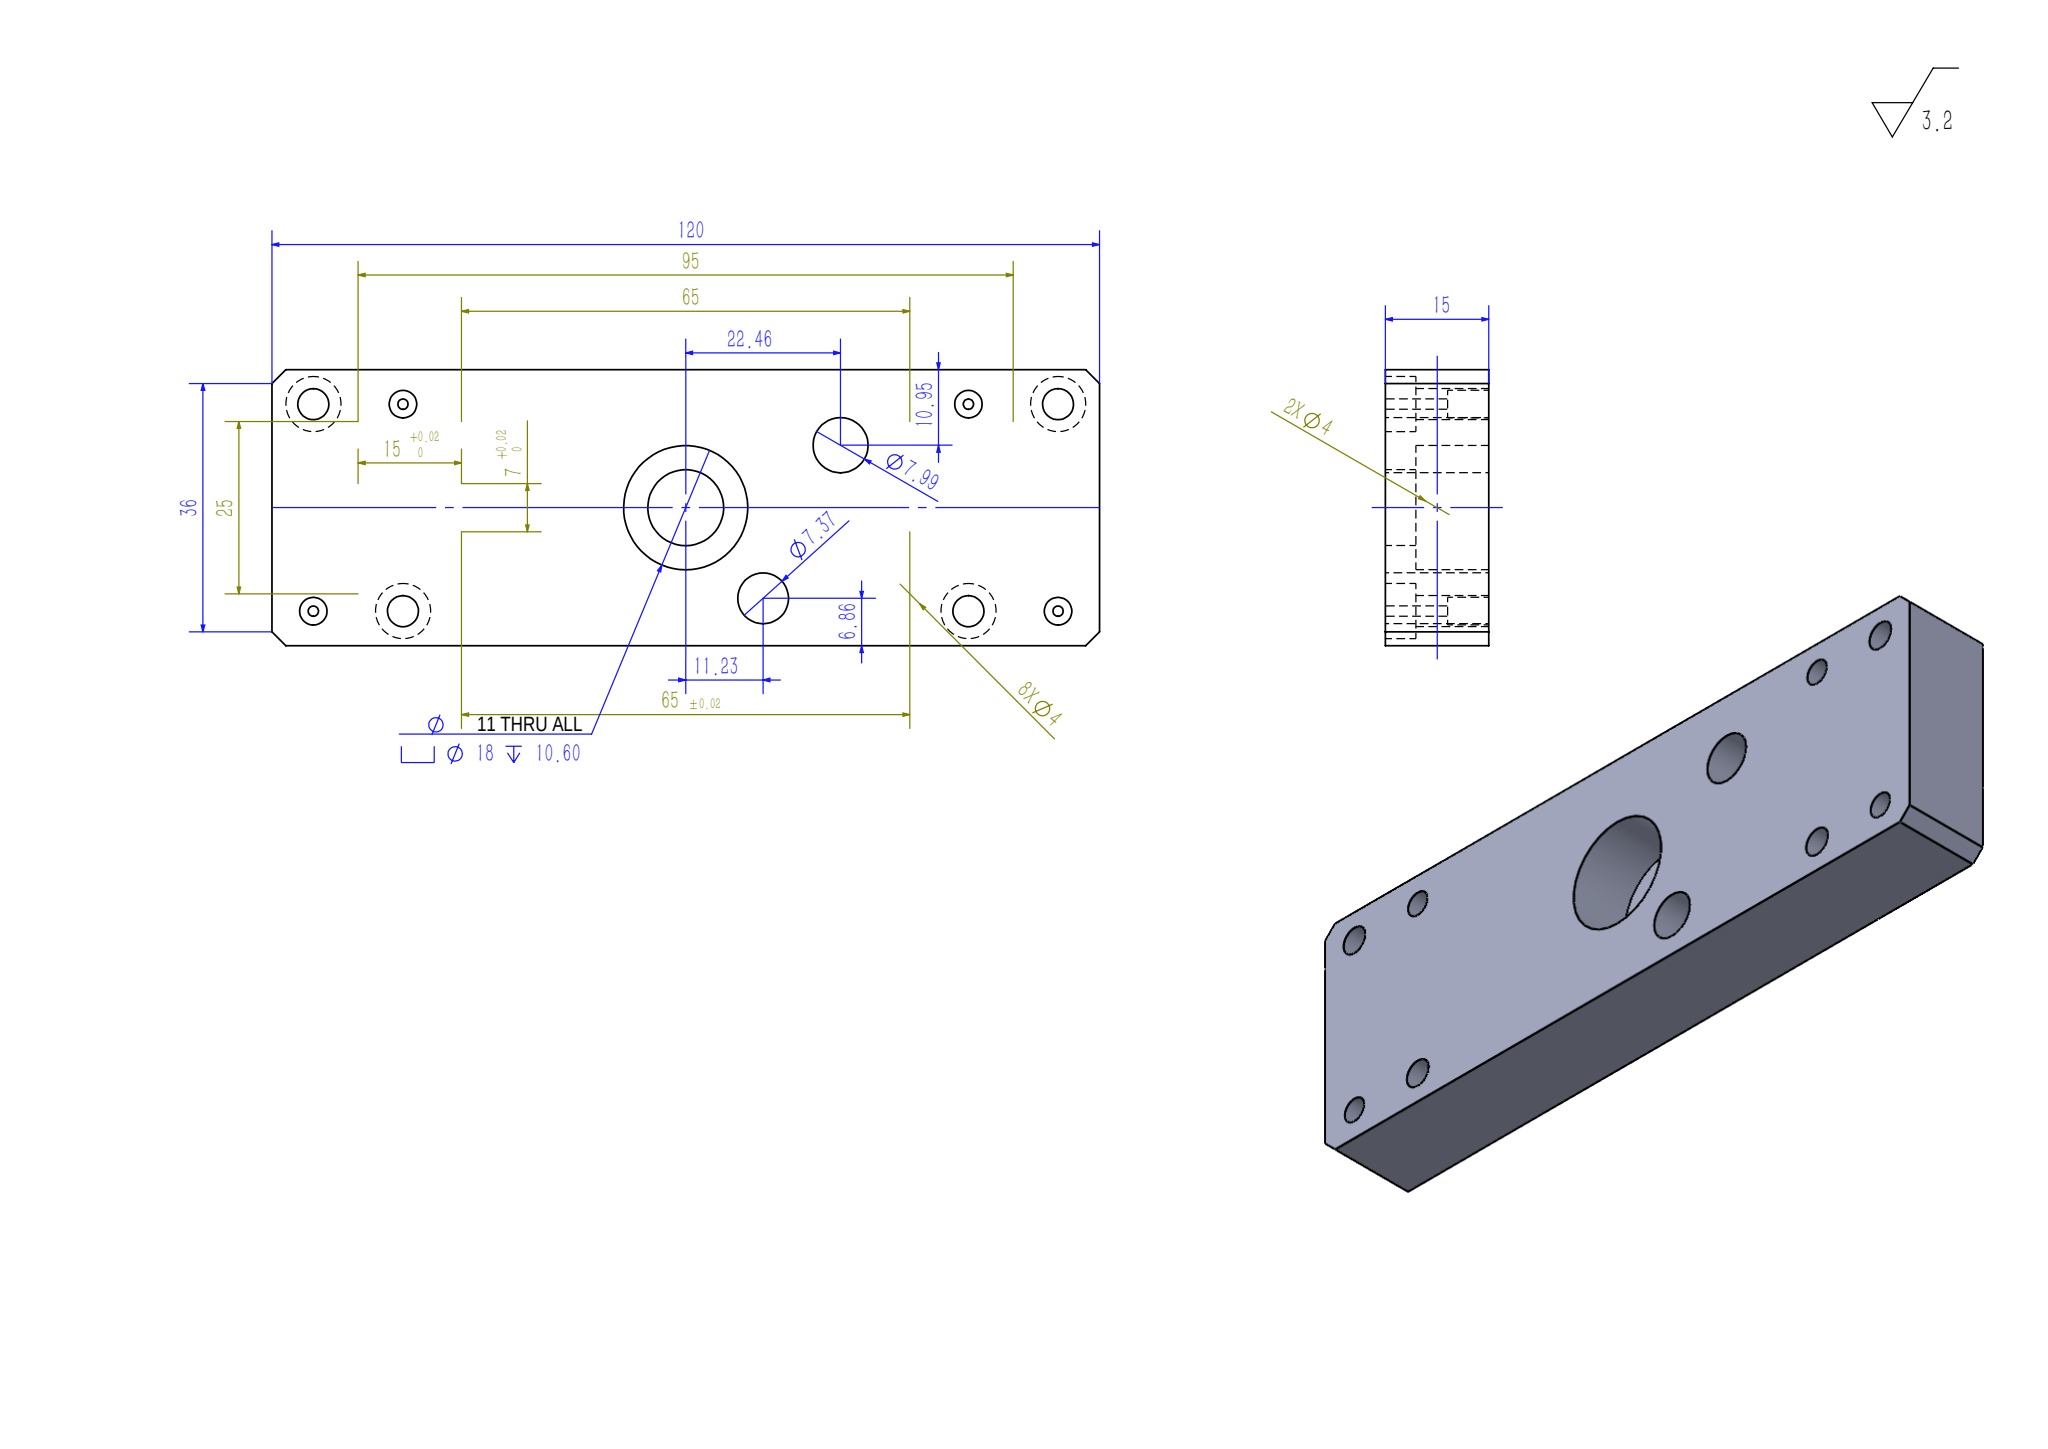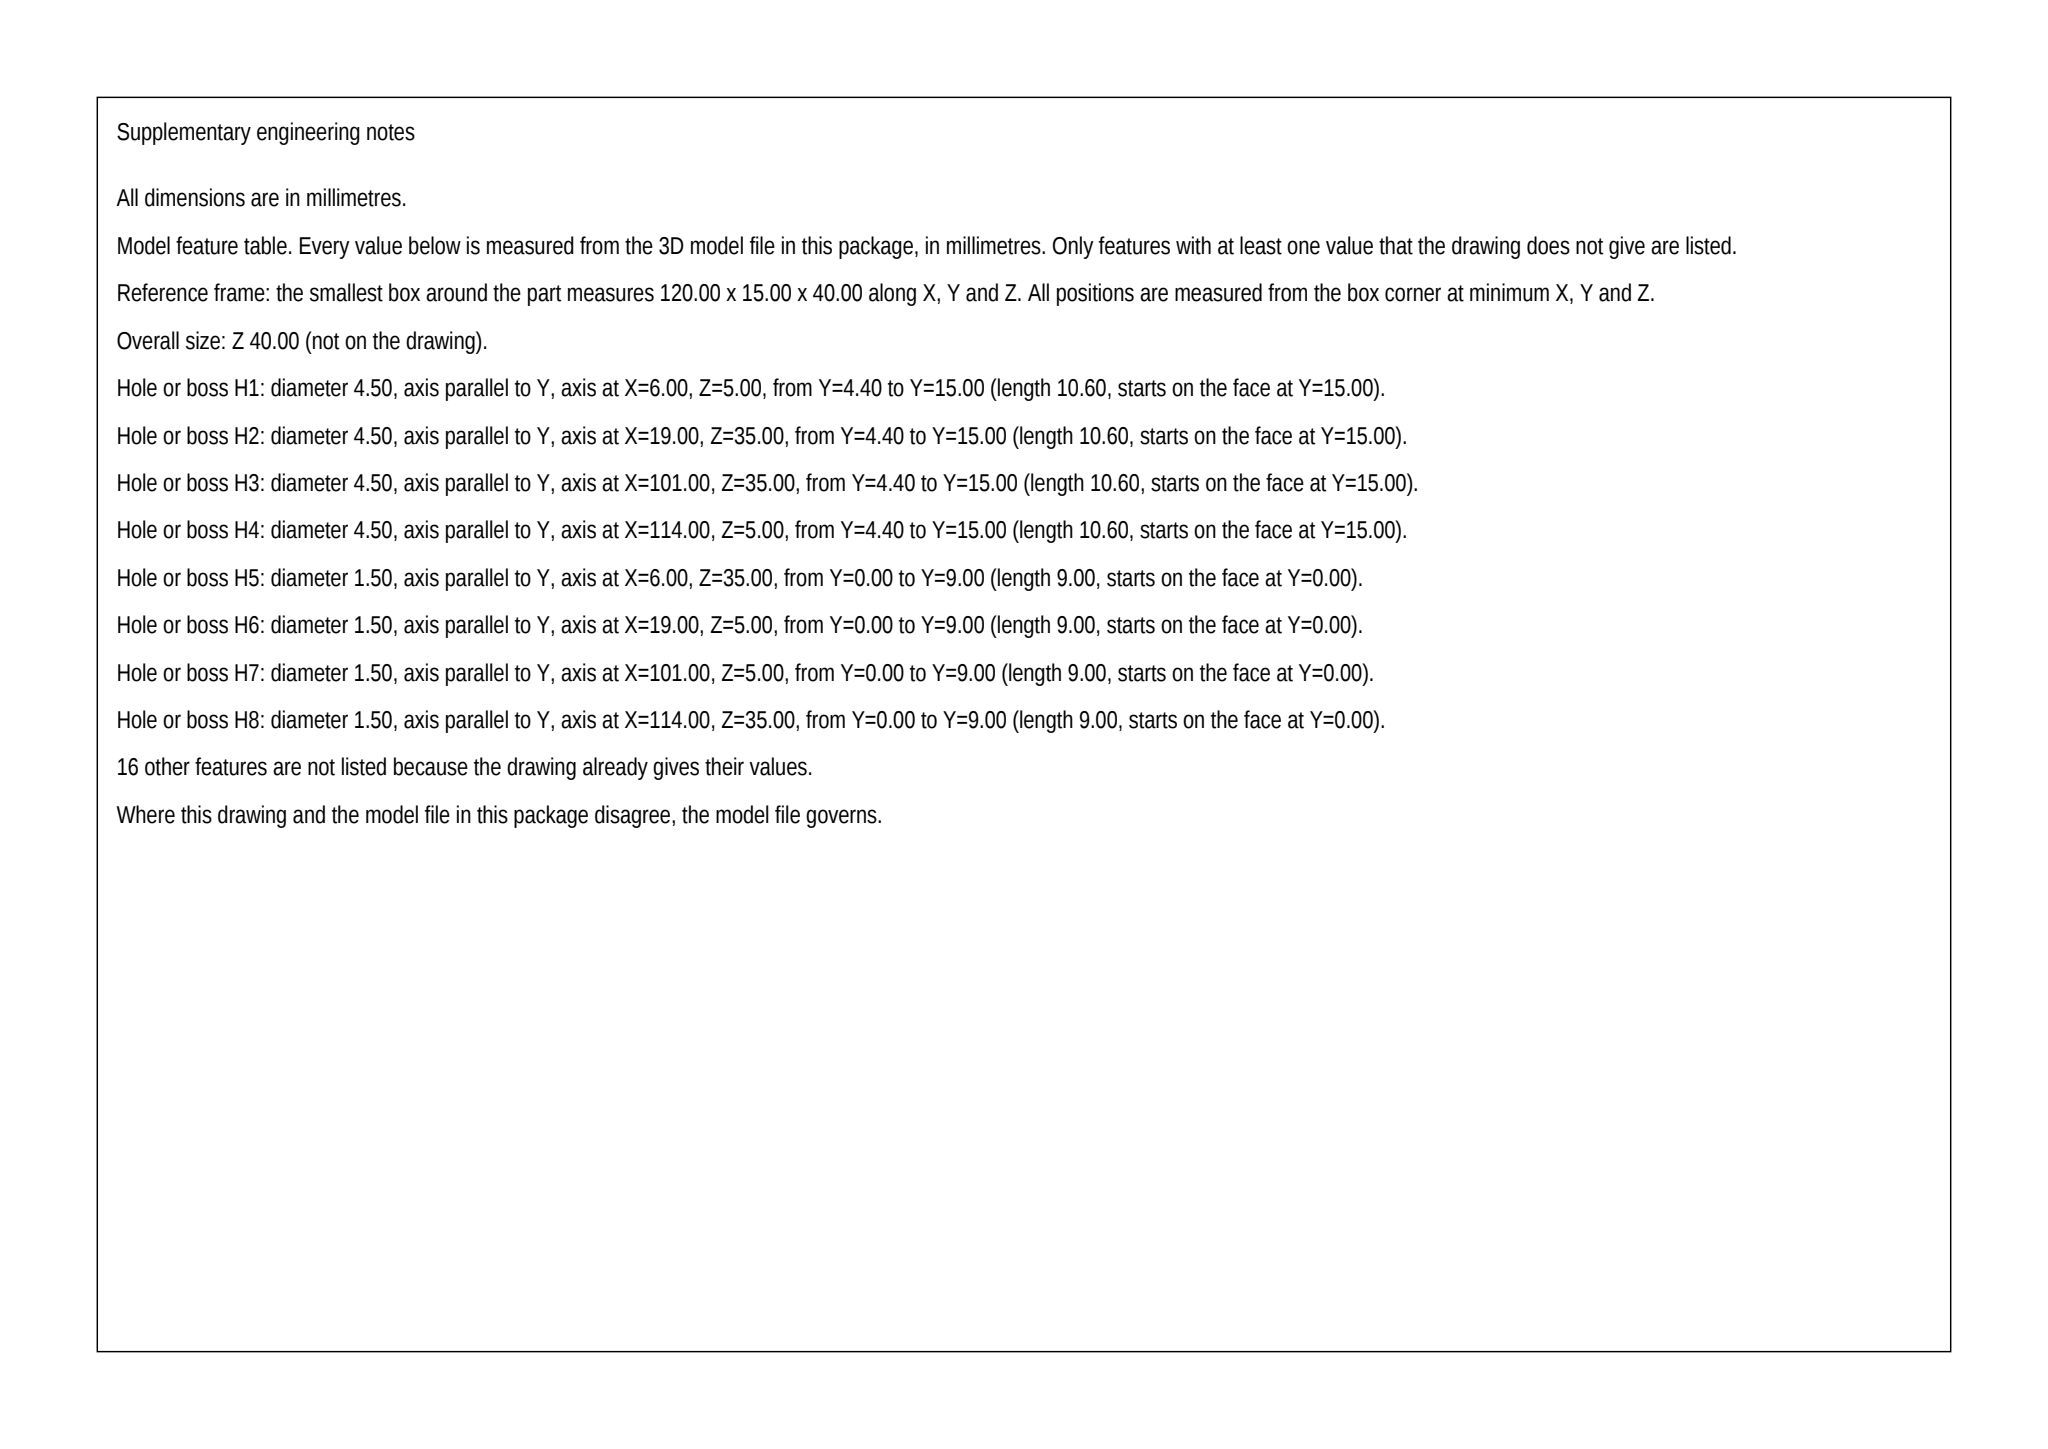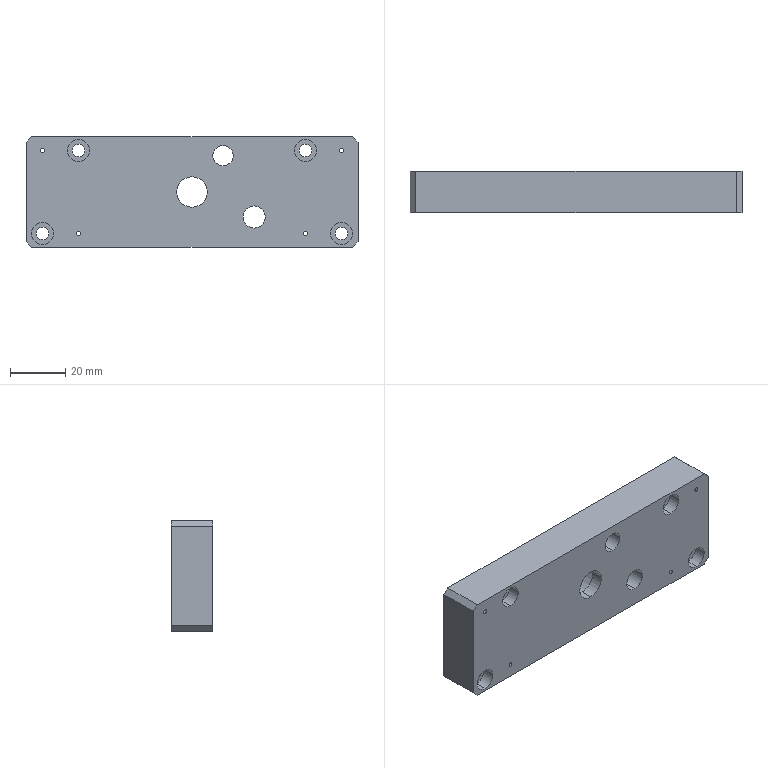Part | SolidWorks | mm | 1 solid | 59 faces | box 120 x 15 x 40 mm | volume 65449 mm3 | cylinder 40 | plane 19 | commonest cylinder face diameters 1.5 x8 4 x8 8 x8 4.5 x8 7.985 x2 7.37 x2 18 x2 11 x2
build123d program:
from build123d import *

# Parameters (mm, degrees)
SKETCH1_W                                        = 120
SKETCH1_H                                        = 40
BOSS_EXTRUDE1_DEPTH                              = 15
M10_HEX_SOCKET_HEAD_CAP_SCREW_CBORE1_D           = 11
M10_HEX_SOCKET_HEAD_CAP_SCREW_CBORE1_CBORE_D     = 18
M10_HEX_SOCKET_HEAD_CAP_SCREW_CBORE1_CBORE_DEPTH = 10.6
M4_HEX_SOCKET_HEAD_CAP_SCREW_CBORE1_AT_2_COUNT   = 2
M4_HEX_SOCKET_HEAD_CAP_SCREW_CBORE1_AT_2_PITCH   = 32.696
SKETCH11_R                                       = 2
CUT_EXTRUDE1_DEPTH                               = 6
CHAMFER1_SIZE                                    = 2
SKETCH12_R                                       = 0.75
CUT_EXTRUDE2_DEPTH                               = 30
SKETCH13_R                                       = 3.993
SKETCH13_R_2                                     = 3.685
CUT_EXTRUDE3_DEPTH                               = 80


with BuildPart() as part:
    # Sketch1 → Boss-Extrude1 (new body)
    with BuildSketch(Plane(origin=(0, 0, 0), x_dir=(1, 0, 0), z_dir=(0, 1, 0))):
        Rectangle(SKETCH1_W, SKETCH1_H)
    extrude(amount=BOSS_EXTRUDE1_DEPTH)

    # M10 Hex Socket Head Cap Screw CBORE1 (through all)
    with Locations(Plane(origin=(0, 15, 0), x_dir=(1, 0, 0), z_dir=(0, 1, 0))):
        with Locations((0, 0)):
            CounterBoreHole(M10_HEX_SOCKET_HEAD_CAP_SCREW_CBORE1_D / 2, M10_HEX_SOCKET_HEAD_CAP_SCREW_CBORE1_CBORE_D / 2, M10_HEX_SOCKET_HEAD_CAP_SCREW_CBORE1_CBORE_DEPTH)

    # Sketch10 → M4 Hex Socket Head Cap Screw CBORE1 (revolve, cut)
    with BuildSketch(Plane(origin=(-41, 0, 15), x_dir=(0, 0, -1), z_dir=(1, 0, 0))):
        Polygon((0, 0), (0, 16.352), (2.25, 15), (2.25, 4.4), (4, 4.4), (4, 0), align=None)
    m4_hex_socket_head_cap_screw_cbore1 = revolve(axis=Axis((-41, -6.35, 15), (0, 1, 0)), mode=Mode.SUBTRACT)

    # M4 Hex Socket Head Cap Screw CBORE1 at 2: M4 Hex Socket Head Cap Screw CBORE1 ×2
    with Locations(*[Vector(-0.3976, 0, -0.9176) * (i * M4_HEX_SOCKET_HEAD_CAP_SCREW_CBORE1_AT_2_PITCH) for i in range(1, M4_HEX_SOCKET_HEAD_CAP_SCREW_CBORE1_AT_2_COUNT)]):
        add(m4_hex_socket_head_cap_screw_cbore1, mode=Mode.SUBTRACT)

    # Sketch11 → Cut-Extrude1 (cut)
    with BuildSketch(Plane(origin=(0, 15, 0), x_dir=(1, 0, 0), z_dir=(0, 1, 0))):
        with Locations(Location((-54, -15, 0), (0, 0, 270))):
            Circle(SKETCH11_R)
        with Locations(Location((-41, 15, 0), (0, 0, 270))):
            Circle(SKETCH11_R)
    cut_extrude1 = extrude(amount=-CUT_EXTRUDE1_DEPTH, mode=Mode.SUBTRACT)

    # Mirror1: M4 Hex Socket Head Cap Screw CBORE1, Cut-Extrude1 across plane
    add(m4_hex_socket_head_cap_screw_cbore1.mirror(Plane(origin=(0, 0, 0), x_dir=(0, 0, 1), z_dir=(1, 0, 0))), mode=Mode.SUBTRACT)
    add(cut_extrude1.mirror(Plane(origin=(0, 0, 0), x_dir=(0, 0, 1), z_dir=(1, 0, 0))), mode=Mode.SUBTRACT)

    # Mirror1 copy 1 sketch → Mirror1 copy 1 (revolve, cut)
    with BuildSketch(Plane(origin=(54, 0, -15), x_dir=(0, 0, -1), z_dir=(-1, 0, 0))):
        Polygon((0, 0), (0, -16.352), (2.25, -15), (2.25, -4.4), (4, -4.4), (4, 0), align=None)
    revolve(axis=Axis((54, -6.35, -15), (0, -1, 0)), mode=Mode.SUBTRACT)

    # Chamfer1
    chamfer1_edges = [part.edges().sort_by_distance(p)[0] for p in [
        (60, 7.5, 20),
        (-60, 7.5, 20),
        (-60, 7.5, -20),
        (60, 7.5, -20),
    ]]
    chamfer(chamfer1_edges, length=CHAMFER1_SIZE)

    # Sketch12 → Cut-Extrude2 (cut)
    with BuildSketch(Plane(origin=(0, 9, 0), x_dir=(1, 0, 0), z_dir=(0, 1, 0))):
        with Locations(Location((-54, -15, 0), (0, 0, 270))):
            Circle(SKETCH12_R)
        with Locations(Location((-41, 15, 0), (0, 0, 270))):
            Circle(SKETCH12_R)
        with Locations(Location((41, 15, 0), (0, 0, 270))):
            Circle(SKETCH12_R)
        with Locations(Location((54, -15, 0), (0, 0, 270))):
            Circle(SKETCH12_R)
    extrude(amount=-CUT_EXTRUDE2_DEPTH, mode=Mode.SUBTRACT)

    # Sketch13 → Cut-Extrude3 (cut)
    with BuildSketch(Plane(origin=(0, 15, 0), x_dir=(1, 0, 0), z_dir=(0, 1, 0))):
        with Locations(Location((22.46, 9.048, 0), (0, 0, 270))):
            Circle(SKETCH13_R)
        with Locations(Location((11.23, -13.138, 0), (0, 0, 270))):
            Circle(SKETCH13_R_2)
    extrude(amount=-CUT_EXTRUDE3_DEPTH, mode=Mode.SUBTRACT)


solid = part.part